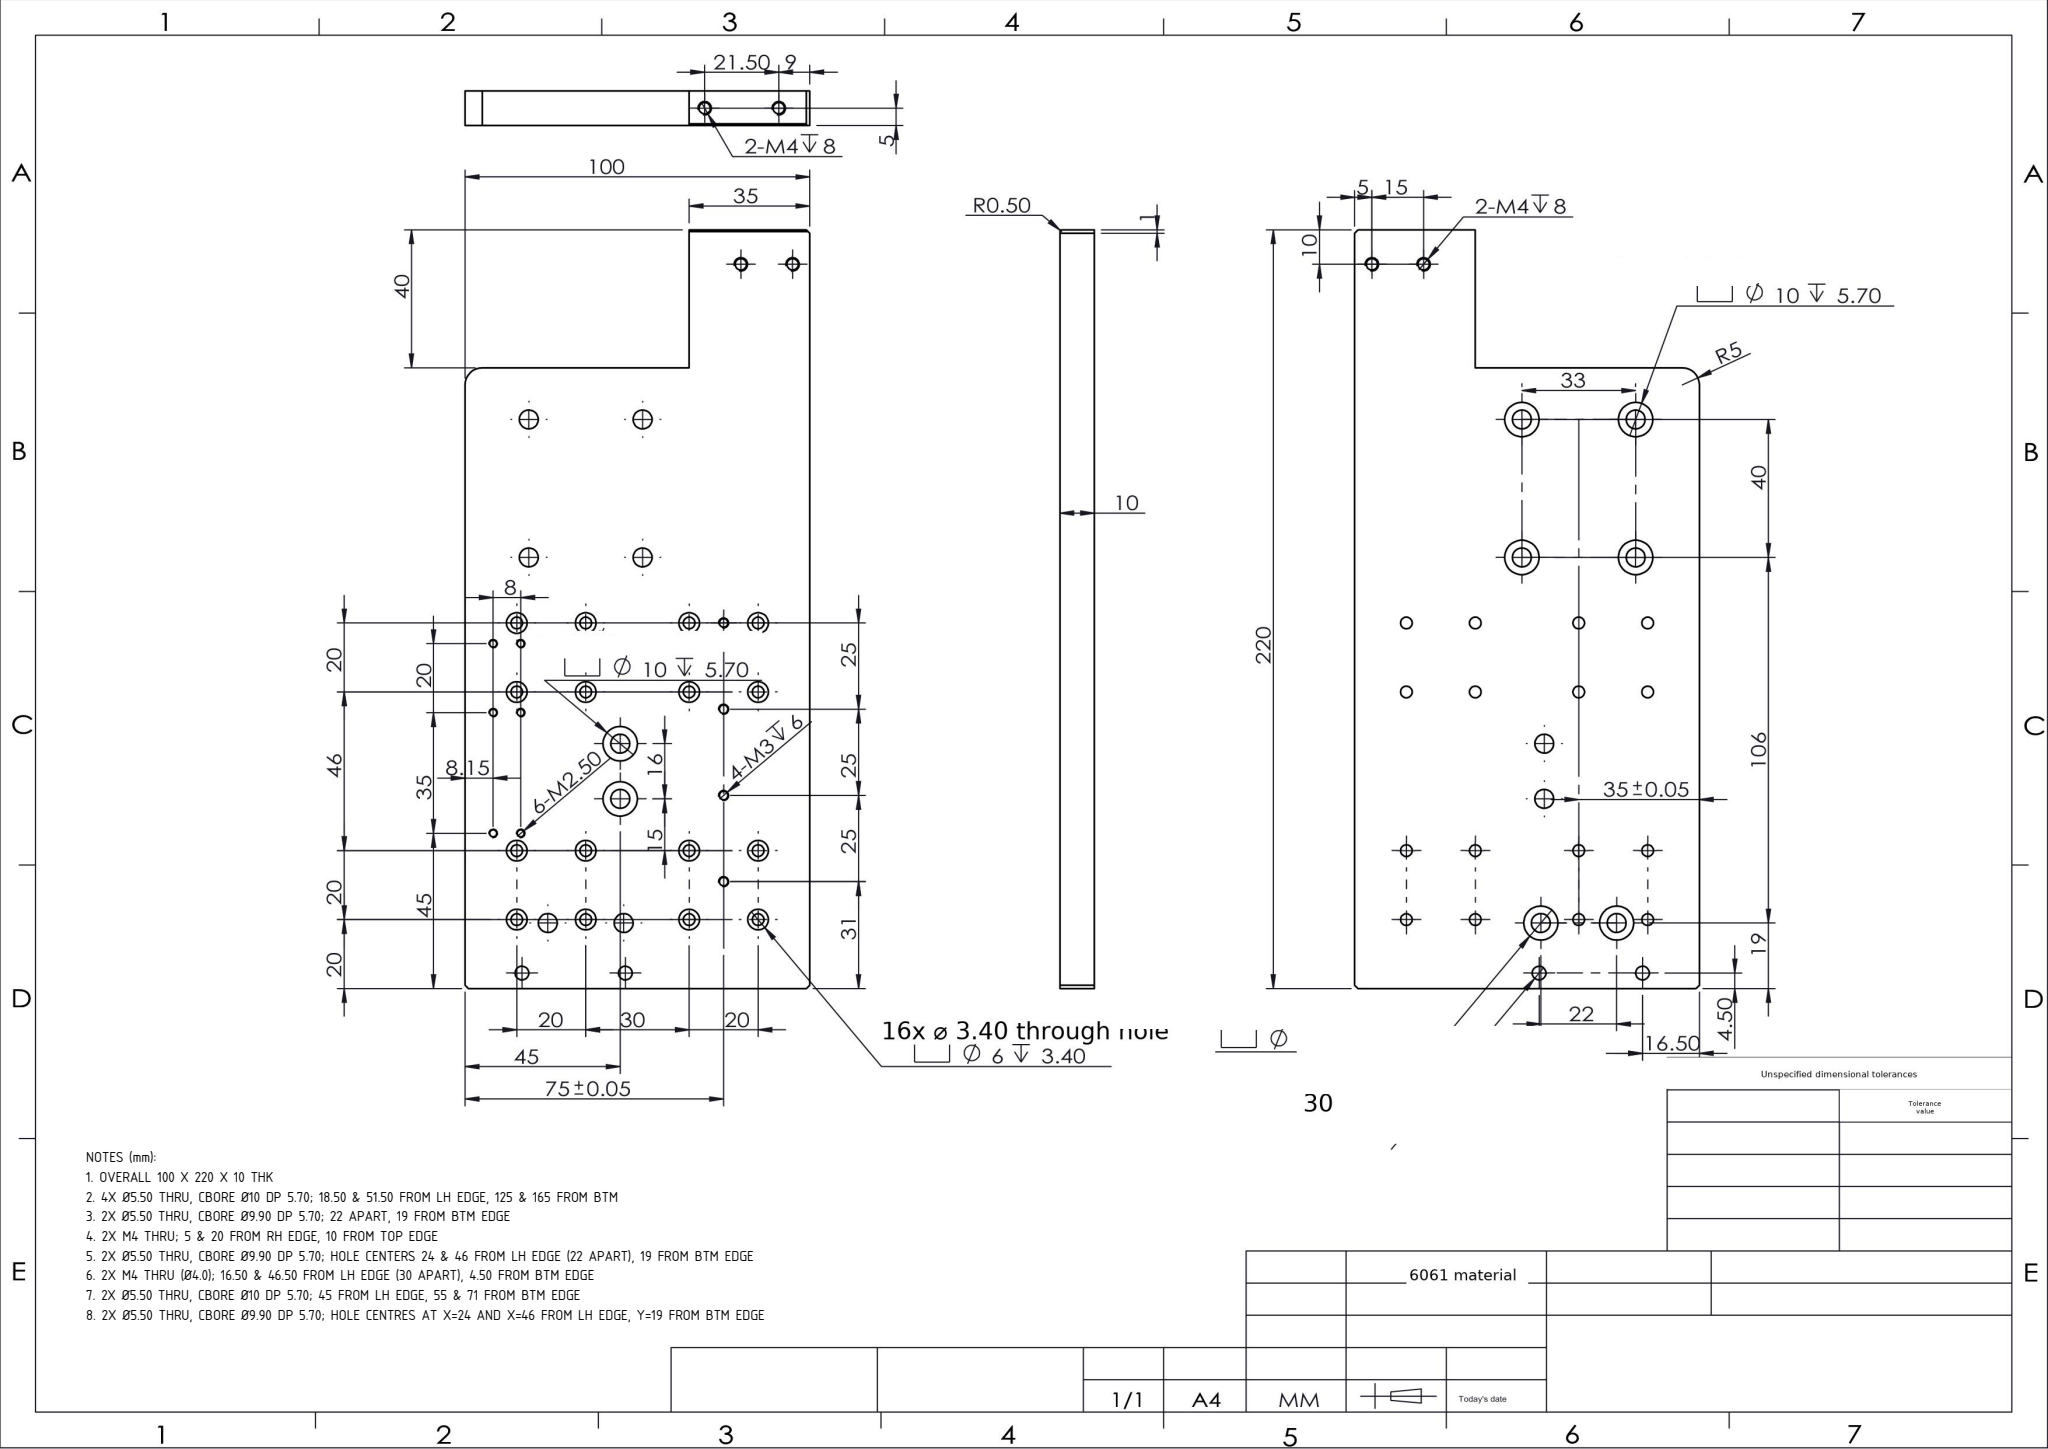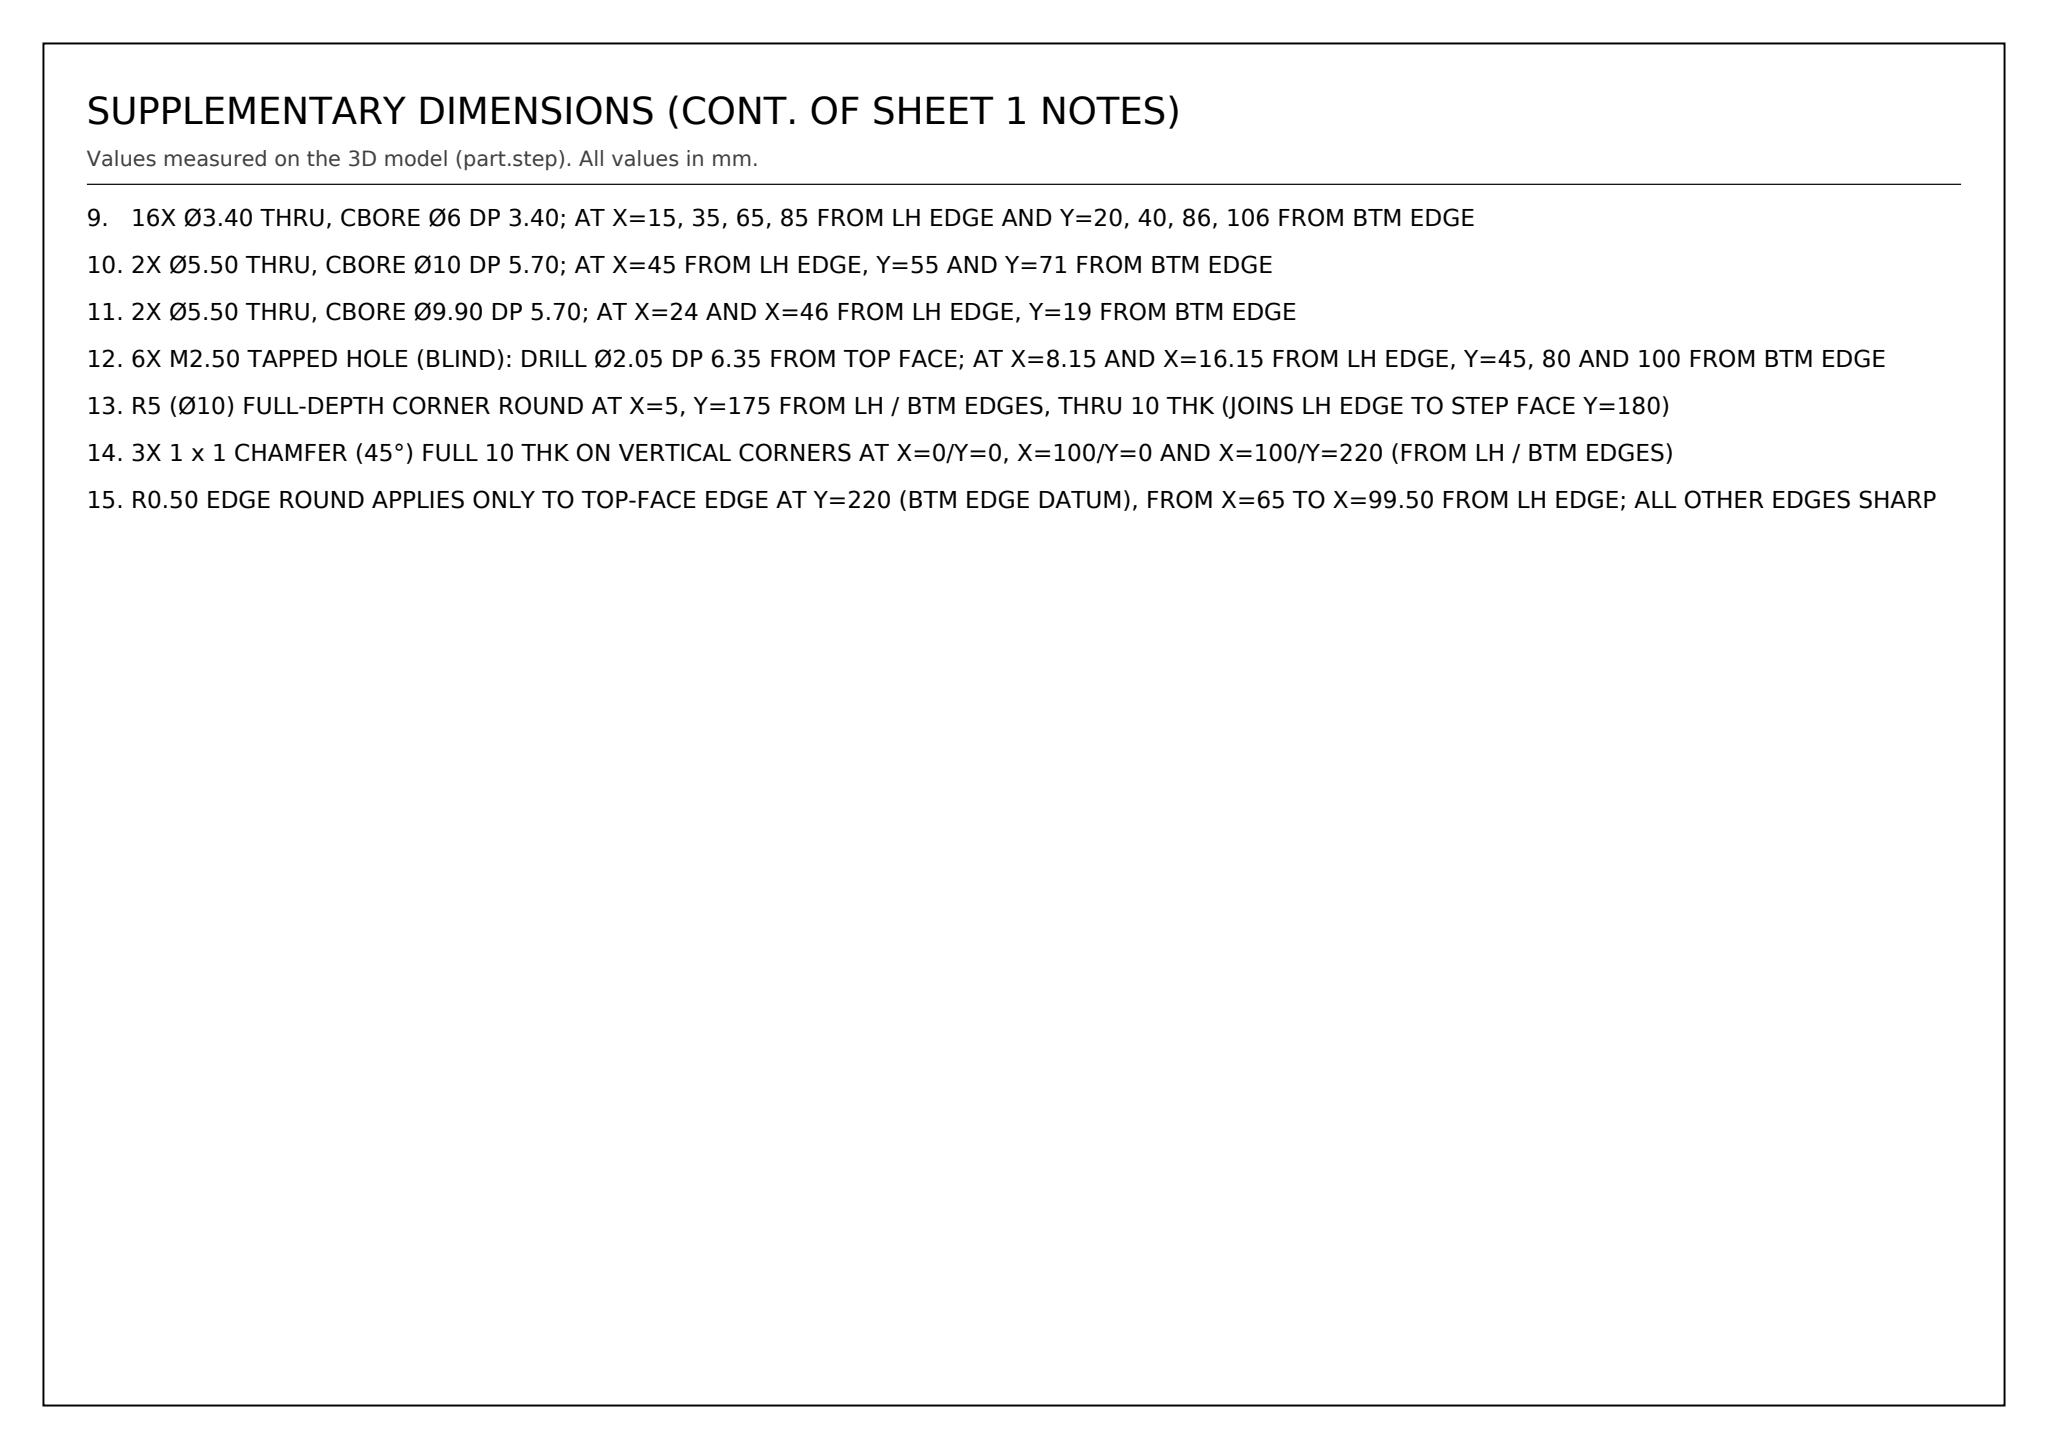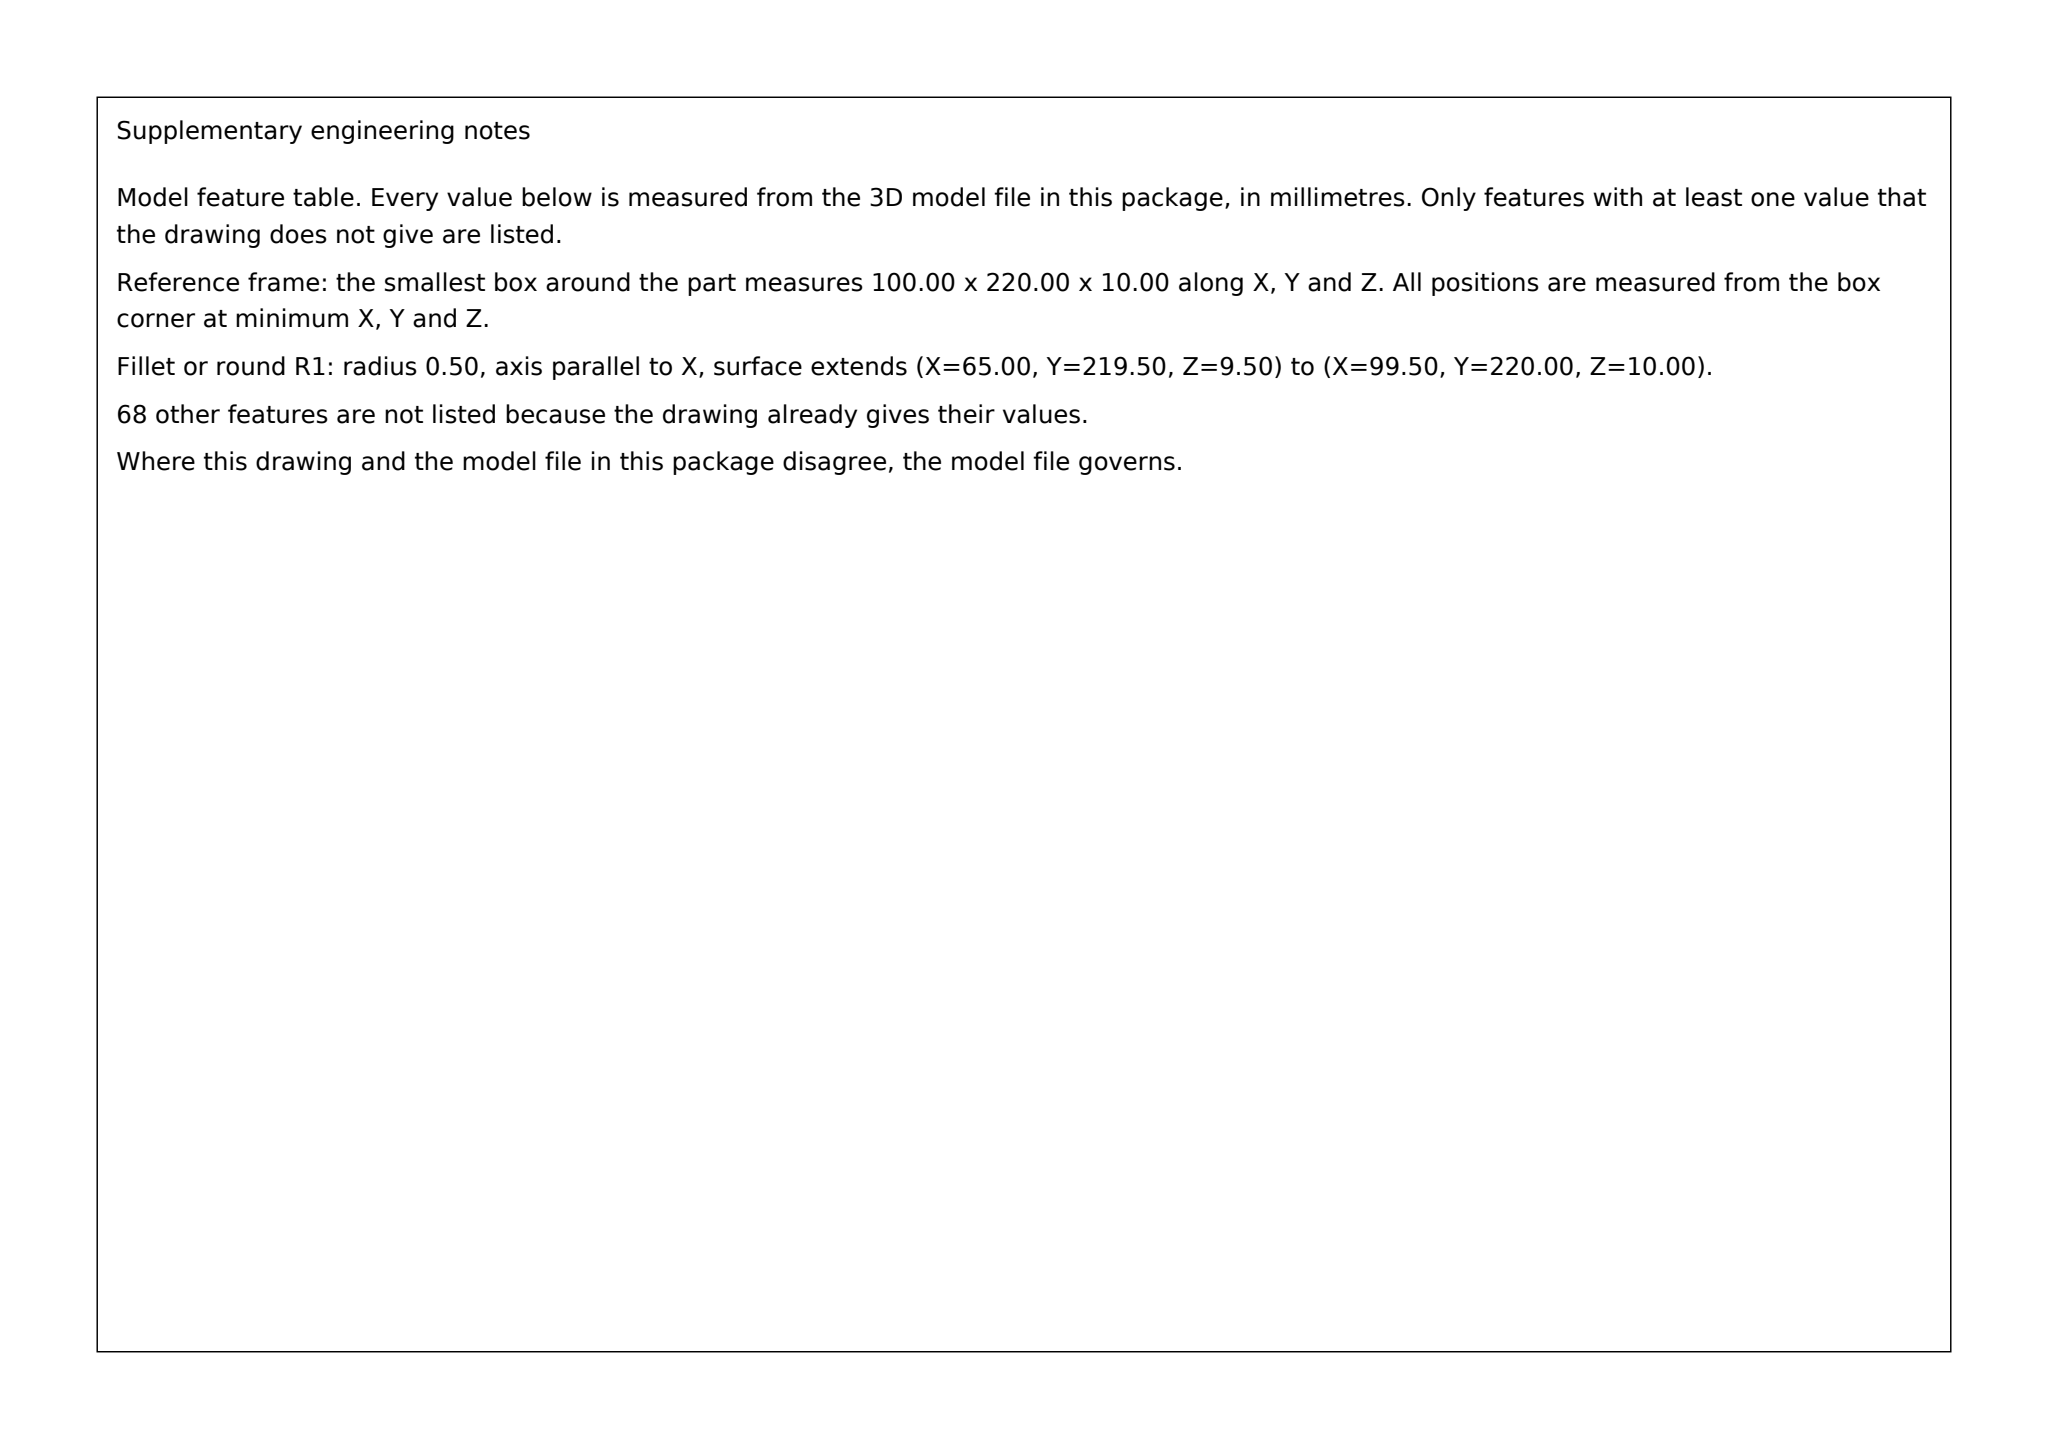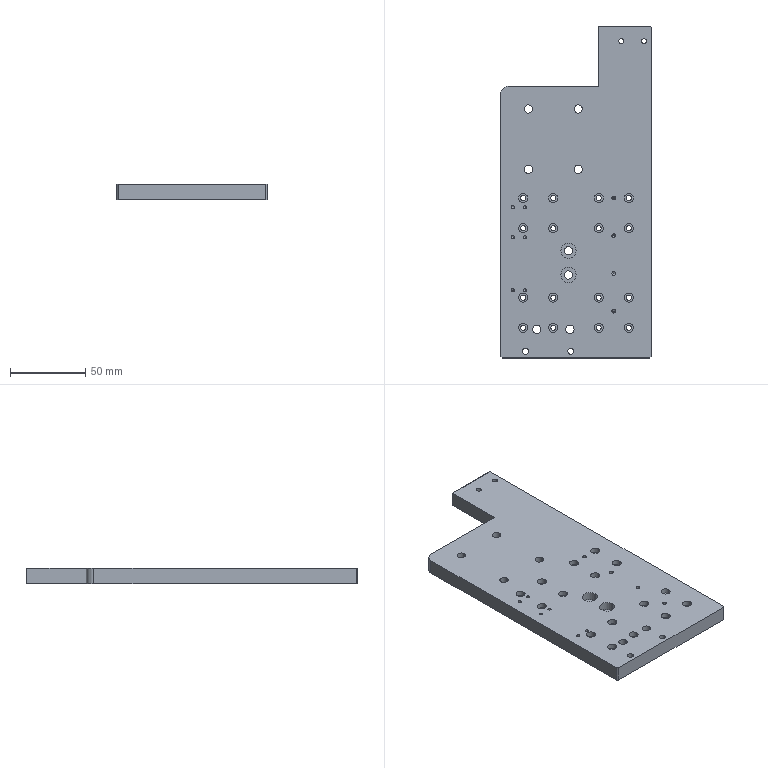Part | SolidWorks | mm | 1 solid | 189 faces | box 100 x 220 x 10 mm | volume 186169 mm3 | cylinder 130 | plane 35 | cone 24 | commonest cylinder face diameters 6 x32 3.4 x32 5.5 x16 10 x13 2.05 x12 2.5 x8 3.3 x8 4 x4
Drawing notes:
OVERALL 100 X 220 X 10 THK | from the solid: bbox_xyz [100.0, 220.0, 10.0]
4X Ø5.50 THRU, CBORE Ø10 DP 5.70; 18.50 & 51.50 FROM LH EDGE, 125 & 165 FROM BTM | from the solid: Ø5.5 thru with Ø10 DP5.70 cbore at (18.5,125),(18.5,165),(51.5,125),(51.5,165); 33 & 40 spacing
2X Ø5.50 THRU, CBORE Ø9.90 DP 5.70; 22 APART, 19 FROM BTM EDGE | from the solid: Ø5.5 thru at (24,19) & (46,19) with Ø9.9 cbore 5.7 deep; spacing 22, y=19
2X M4 THRU; 5 & 20 FROM RH EDGE, 10 FROM TOP EDGE | from the solid: Ø3.3 z-axis holes thru 10 thk at (80,210) & (95,210); 100-95=5, 100-80=20, 220-210=10
2X Ø5.50 THRU, CBORE Ø9.90 DP 5.70; HOLE CENTERS 24 & 46 FROM LH EDGE (22 APART), 19 FROM BTM EDGE | from the solid: cylinders dia 5.5 axis z at [24,19] and [46,19] len 4.3, with dia 9.9 axis z at [24,19] and [46,19] len 5.7
2X M4 THRU (Ø4.0); 16.50 & 46.50 FROM LH EDGE (30 APART), 4.50 FROM BTM EDGE | from the solid: cylinders dia 4.0 axis z at [16.5,4.5] and [46.5,4.5] len 10.0 (full 10 thk)
2X Ø5.50 THRU, CBORE Ø10 DP 5.70; 45 FROM LH EDGE, 55 & 71 FROM BTM EDGE | from the solid: cylinders dia 5.5 axis z at [45,55] and [45,71] len 4.3, with dia 10.0 axis z at same positions len 5.7
2X Ø5.50 THRU, CBORE Ø9.90 DP 5.70; HOLE CENTRES AT X=24 AND X=46 FROM LH EDGE, Y=19 FROM BTM EDGE | from the solid: cylinders dia 5.5 z-axis at (24,19) and (46,19) len 4.3 with dia 9.9 z-axis counterbores at same XY, len 5.7
16X Ø3.40 THRU, CBORE Ø6 DP 3.40; AT X=15, 35, 65, 85 FROM LH EDGE AND Y=20, 40, 86, 106 FROM BTM EDGE | from the solid: cylinders dia 3.4 z-axis len 6.6 at x=15/35/65/85, y=20/40/86/106 with dia 6.0 counterbores len 3.4 at same XY
2X Ø5.50 THRU, CBORE Ø10 DP 5.70; AT X=45 FROM LH EDGE, Y=55 AND Y=71 FROM BTM EDGE | from the solid: cylinders dia 5.5 z-axis at (45,55) and (45,71) len 4.3 with dia 10.0 counterbores len 5.7 at same XY
2X Ø5.50 THRU, CBORE Ø9.90 DP 5.70; AT X=24 AND X=46 FROM LH EDGE, Y=19 FROM BTM EDGE | from the solid: Ø5.5 z-cylinders at (24,19) and (46,19) with coaxial Ø9.9 z-cylinders L=5.7 at (24,19) and (46,19)
6X M2.50 TAPPED HOLE (BLIND): DRILL Ø2.05 DP 6.35 FROM TOP FACE; AT X=8.15 AND X=16.15 FROM LH EDGE, Y=45, 80 AND 100 FROM BTM EDGE | from the solid: cylinders dia 2.05, axis z, length 6.35 at (8.15,45),(8.15,80),(8.15,100),(16.15,45),(16.15,80),(16.15,100); cones 118deg ref_dia 2.05 (drill points)
R5 (Ø10) FULL-DEPTH CORNER ROUND AT X=5, Y=175 FROM LH / BTM EDGES, THRU 10 THK (JOINS LH EDGE TO STEP FACE Y=180) | from the solid: cylinders: convex arc (round/outer radius) dia 10.0, axis z at [5.0, 175.0], from z=0.0 to 10.0, arc_deg 90; planes x=0 extent y[1,175] and y=180 extent x[5,65]
3X 1 x 1 CHAMFER (45°) FULL 10 THK ON VERTICAL CORNERS AT X=0/Y=0, X=100/Y=0 AND X=100/Y=220 (FROM LH / BTM EDGES) | from the solid: inclined_planes: three 45°/45° faces, size [1.0,1.0,10.0] at bbox_from [0,0,0], [99,0,0], [99,219,0]
R0.50 EDGE ROUND APPLIES ONLY TO TOP-FACE EDGE AT Y=220 (BTM EDGE DATUM), FROM X=65 TO X=99.50 FROM LH EDGE; ALL OTHER EDGES SHARP | from the solid: cylinders: convex arc (round/outer radius) dia 1.0, axis x at (y=219.5, z=9.5), from x=65.0 to x=99.5, 90°
build123d program:
from build123d import *

# Parameters (mm, degrees)
SKETCH1_W                                            = 100
SKETCH1_H                                            = 120
BOSS_EXTRUDE1_DEPTH                                  = 10
HOLE_SIZE_ACCORDING_TO_THE_TYPE_OF_HEXAG_D           = 3.4
HOLE_SIZE_ACCORDING_TO_THE_TYPE_OF_HEXAG_CBORE_D     = 6
HOLE_SIZE_ACCORDING_TO_THE_TYPE_OF_HEXAG_CBORE_DEPTH = 3.4
LPATTERN1_COUNT                                      = 2
LPATTERN1_PITCH                                      = 20
LPATTERN2_COUNT                                      = 2
LPATTERN2_PITCH                                      = 66
LPATTERN2_COPY_1_D                                   = 3.4
LPATTERN2_COPY_1_CBORE_D                             = 6
LPATTERN2_COPY_1_CBORE_DEPTH                         = 3.4
CHAMFER1_SIZE                                        = 1
BOSS_EXTRUDE2_DEPTH                                  = 10
HOLE_SIZE_ACCORDING_TO_THE_TYPE_OF_H_2_D             = 5.5
HOLE_SIZE_ACCORDING_TO_THE_TYPE_OF_H_2_CBORE_D       = 10
HOLE_SIZE_ACCORDING_TO_THE_TYPE_OF_H_2_CBORE_DEPTH   = 5.7
HOLE_SIZE_ACCORDING_TO_THE_TYPE_OF_H_3_D             = 5.5
HOLE_SIZE_ACCORDING_TO_THE_TYPE_OF_H_3_CBORE_D       = 10
HOLE_SIZE_ACCORDING_TO_THE_TYPE_OF_H_3_CBORE_DEPTH   = 5.7
M4_TAPPED_HOLE3_D                                    = 3.3
M4_TAPPED_HOLE3_DEPTH                                = 10.1
M4_TAPPED_HOLE3_TIP                                  = 0.9914
HOLE_SIZE_ACCORDING_TO_THE_TYPE_OF_H_4_D             = 5.5
HOLE_SIZE_ACCORDING_TO_THE_TYPE_OF_H_4_CBORE_D       = 9.9
HOLE_SIZE_ACCORDING_TO_THE_TYPE_OF_H_4_CBORE_DEPTH   = 5.7
SKETCH28_R                                           = 2
CUT_EXTRUDE2_DEPTH                                   = 10
M2_5_TAPPED_HOLE2_D                                  = 2.05
M2_5_TAPPED_HOLE2_DEPTH                              = 6.35
M2_5_TAPPED_HOLE2_TIP                                = 0.6159
CHAMFER2_SIZE                                        = 1
M4_TAPPED_HOLE4_D                                    = 3.3
M4_TAPPED_HOLE4_DEPTH                                = 10.1
M4_TAPPED_HOLE4_TIP                                  = 0.9914
FILLET1_R                                            = 0.5
FILLET2_R                                            = 5
LPATTERN4_COUNT                                      = 4
LPATTERN4_PITCH                                      = 25


with BuildPart() as part:
    # Sketch1 → Boss-Extrude1 (new body)
    with BuildSketch(Plane.XY):
        with Locations((50, 60)):
            Rectangle(SKETCH1_W, SKETCH1_H)
    extrude(amount=BOSS_EXTRUDE1_DEPTH)

    # Hole Size according to the type of Hexag (through all)
    with Locations(Plane.XY.offset(10)):
        with Locations((15, 20), (35, 20), (65, 20), (85, 20)):
            hole_size_according_to_the_type_of_hexag = CounterBoreHole(HOLE_SIZE_ACCORDING_TO_THE_TYPE_OF_HEXAG_D / 2, HOLE_SIZE_ACCORDING_TO_THE_TYPE_OF_HEXAG_CBORE_D / 2, HOLE_SIZE_ACCORDING_TO_THE_TYPE_OF_HEXAG_CBORE_DEPTH)

    # LPattern1: Hole Size according to the type of Hexag ×2
    with Locations(*[(0, i * LPATTERN1_PITCH, 0) for i in range(1, LPATTERN1_COUNT)]):
        add(hole_size_according_to_the_type_of_hexag, mode=Mode.SUBTRACT)

    # LPattern2: Hole Size according to the type of Hexag ×2
    with Locations(*[(0, i * LPATTERN2_PITCH, 0) for i in range(1, LPATTERN2_COUNT)]):
        add(hole_size_according_to_the_type_of_hexag, mode=Mode.SUBTRACT)

    # LPattern2 copy 1 (through all)
    with Locations(Plane(origin=(0, 86, 10), x_dir=(1, 0, 0), z_dir=(0, 0, 1))):
        with Locations((15, 20), (35, 20), (65, 20), (85, 20)):
            CounterBoreHole(LPATTERN2_COPY_1_D / 2, LPATTERN2_COPY_1_CBORE_D / 2, LPATTERN2_COPY_1_CBORE_DEPTH)

    # Chamfer1
    chamfer1_edges = [part.edges().sort_by_distance(p)[0] for p in [
        (100, 0, 5),
        (0, 0, 5),
    ]]
    chamfer(chamfer1_edges, length=CHAMFER1_SIZE)

    # Sketch12 → M3 Tapped Hole1 (revolve, cut)
    with BuildSketch(Plane(origin=(75, 106, 10), x_dir=(0, -1, 0), z_dir=(1, 0, 0))):
        Polygon((0, 0), (0, 8.251), (1.25, 7.5), (1.25, 0), align=None)
    m3_tapped_hole1 = revolve(axis=Axis((75, 106, 16.35), (0, 0, -1)), mode=Mode.SUBTRACT)

    # Sketch15 → Boss-Extrude2 (add)
    with BuildSketch(Plane.XY.offset(10)):
        Polygon((65, 180), (65, 220), (100, 220), (100, 114), (0, 114), (0, 180), align=None)
    extrude(amount=-BOSS_EXTRUDE2_DEPTH)

    # Hole Size according to the type of H 2 (through all)
    with Locations(Plane(origin=(0, 0, 0), x_dir=(-1, 0, 0), z_dir=(0, 0, -1))):
        with Locations((-51.5, 165), (-18.5, 165), (-51.5, 125), (-18.5, 125)):
            CounterBoreHole(HOLE_SIZE_ACCORDING_TO_THE_TYPE_OF_H_2_D / 2, HOLE_SIZE_ACCORDING_TO_THE_TYPE_OF_H_2_CBORE_D / 2, HOLE_SIZE_ACCORDING_TO_THE_TYPE_OF_H_2_CBORE_DEPTH)

    # Hole Size according to the type of H 3 (through all)
    with Locations(Plane.XY.offset(10)):
        with Locations((45, 71), (45, 55)):
            CounterBoreHole(HOLE_SIZE_ACCORDING_TO_THE_TYPE_OF_H_3_D / 2, HOLE_SIZE_ACCORDING_TO_THE_TYPE_OF_H_3_CBORE_D / 2, HOLE_SIZE_ACCORDING_TO_THE_TYPE_OF_H_3_CBORE_DEPTH)

    # M4 Tapped Hole3
    with Locations(Plane(origin=(0, 0, 0), x_dir=(-1, 0, 0), z_dir=(0, 0, -1))):
        with Locations((-95, 210), (-80, 210)):
            Hole(M4_TAPPED_HOLE3_D / 2, depth=M4_TAPPED_HOLE3_DEPTH)
            with Locations((0, 0, -(M4_TAPPED_HOLE3_DEPTH + M4_TAPPED_HOLE3_TIP / 2))):  # 118° drill point
                Cone(0, M4_TAPPED_HOLE3_D / 2, M4_TAPPED_HOLE3_TIP, mode=Mode.SUBTRACT)

    # Hole Size according to the type of H 4 (through all)
    with Locations(Plane(origin=(0, 0, 0), x_dir=(-1, 0, 0), z_dir=(0, 0, -1))):
        with Locations((-24, 19), (-46, 19)):
            CounterBoreHole(HOLE_SIZE_ACCORDING_TO_THE_TYPE_OF_H_4_D / 2, HOLE_SIZE_ACCORDING_TO_THE_TYPE_OF_H_4_CBORE_D / 2, HOLE_SIZE_ACCORDING_TO_THE_TYPE_OF_H_4_CBORE_DEPTH)

    # Sketch28 → Cut-Extrude2 (cut)
    with BuildSketch(Plane.XY.offset(10)):
        with Locations((16.5, 4.5)):
            Circle(SKETCH28_R)
        with Locations((46.5, 4.5)):
            Circle(SKETCH28_R)
    extrude(amount=-CUT_EXTRUDE2_DEPTH, mode=Mode.SUBTRACT)

    # M2.5 Tapped Hole2
    with Locations(Plane.XY.offset(10)):
        with Locations((8.146, 100), (16.146, 100), (8.146, 80), (16.146, 80), (8.146, 45), (16.146, 45)):
            Hole(M2_5_TAPPED_HOLE2_D / 2, depth=M2_5_TAPPED_HOLE2_DEPTH)
            with Locations((0, 0, -(M2_5_TAPPED_HOLE2_DEPTH + M2_5_TAPPED_HOLE2_TIP / 2))):  # 118° drill point
                Cone(0, M2_5_TAPPED_HOLE2_D / 2, M2_5_TAPPED_HOLE2_TIP, mode=Mode.SUBTRACT)

    # Chamfer2
    chamfer2_edges = [part.edges().sort_by_distance(p)[0] for p in [
        (100, 220, 5),
    ]]
    chamfer(chamfer2_edges, length=CHAMFER2_SIZE)

    # M4 Tapped Hole4
    with Locations(Plane(origin=(0, 220, 0), x_dir=(1, 0, 0), z_dir=(0, 1, 0))):
        with Locations((69.5, -5), (91, -5)):
            Hole(M4_TAPPED_HOLE4_D / 2, depth=M4_TAPPED_HOLE4_DEPTH)
            with Locations((0, 0, -(M4_TAPPED_HOLE4_DEPTH + M4_TAPPED_HOLE4_TIP / 2))):  # 118° drill point
                Cone(0, M4_TAPPED_HOLE4_D / 2, M4_TAPPED_HOLE4_TIP, mode=Mode.SUBTRACT)

    # Fillet1
    fillet1_edges = [part.edges().sort_by_distance(p)[0] for p in [
        (82, 220, 10),
    ]]
    fillet(fillet1_edges, radius=FILLET1_R)

    # Fillet2
    fillet2_edges = [part.edges().sort_by_distance(p)[0] for p in [
        (0, 180, 5),
    ]]
    fillet(fillet2_edges, radius=FILLET2_R)

    # LPattern4: M3 Tapped Hole1 ×4
    with Locations(*[(0, -i * LPATTERN4_PITCH, 0) for i in range(1, LPATTERN4_COUNT)]):
        add(m3_tapped_hole1, mode=Mode.SUBTRACT)


solid = part.part